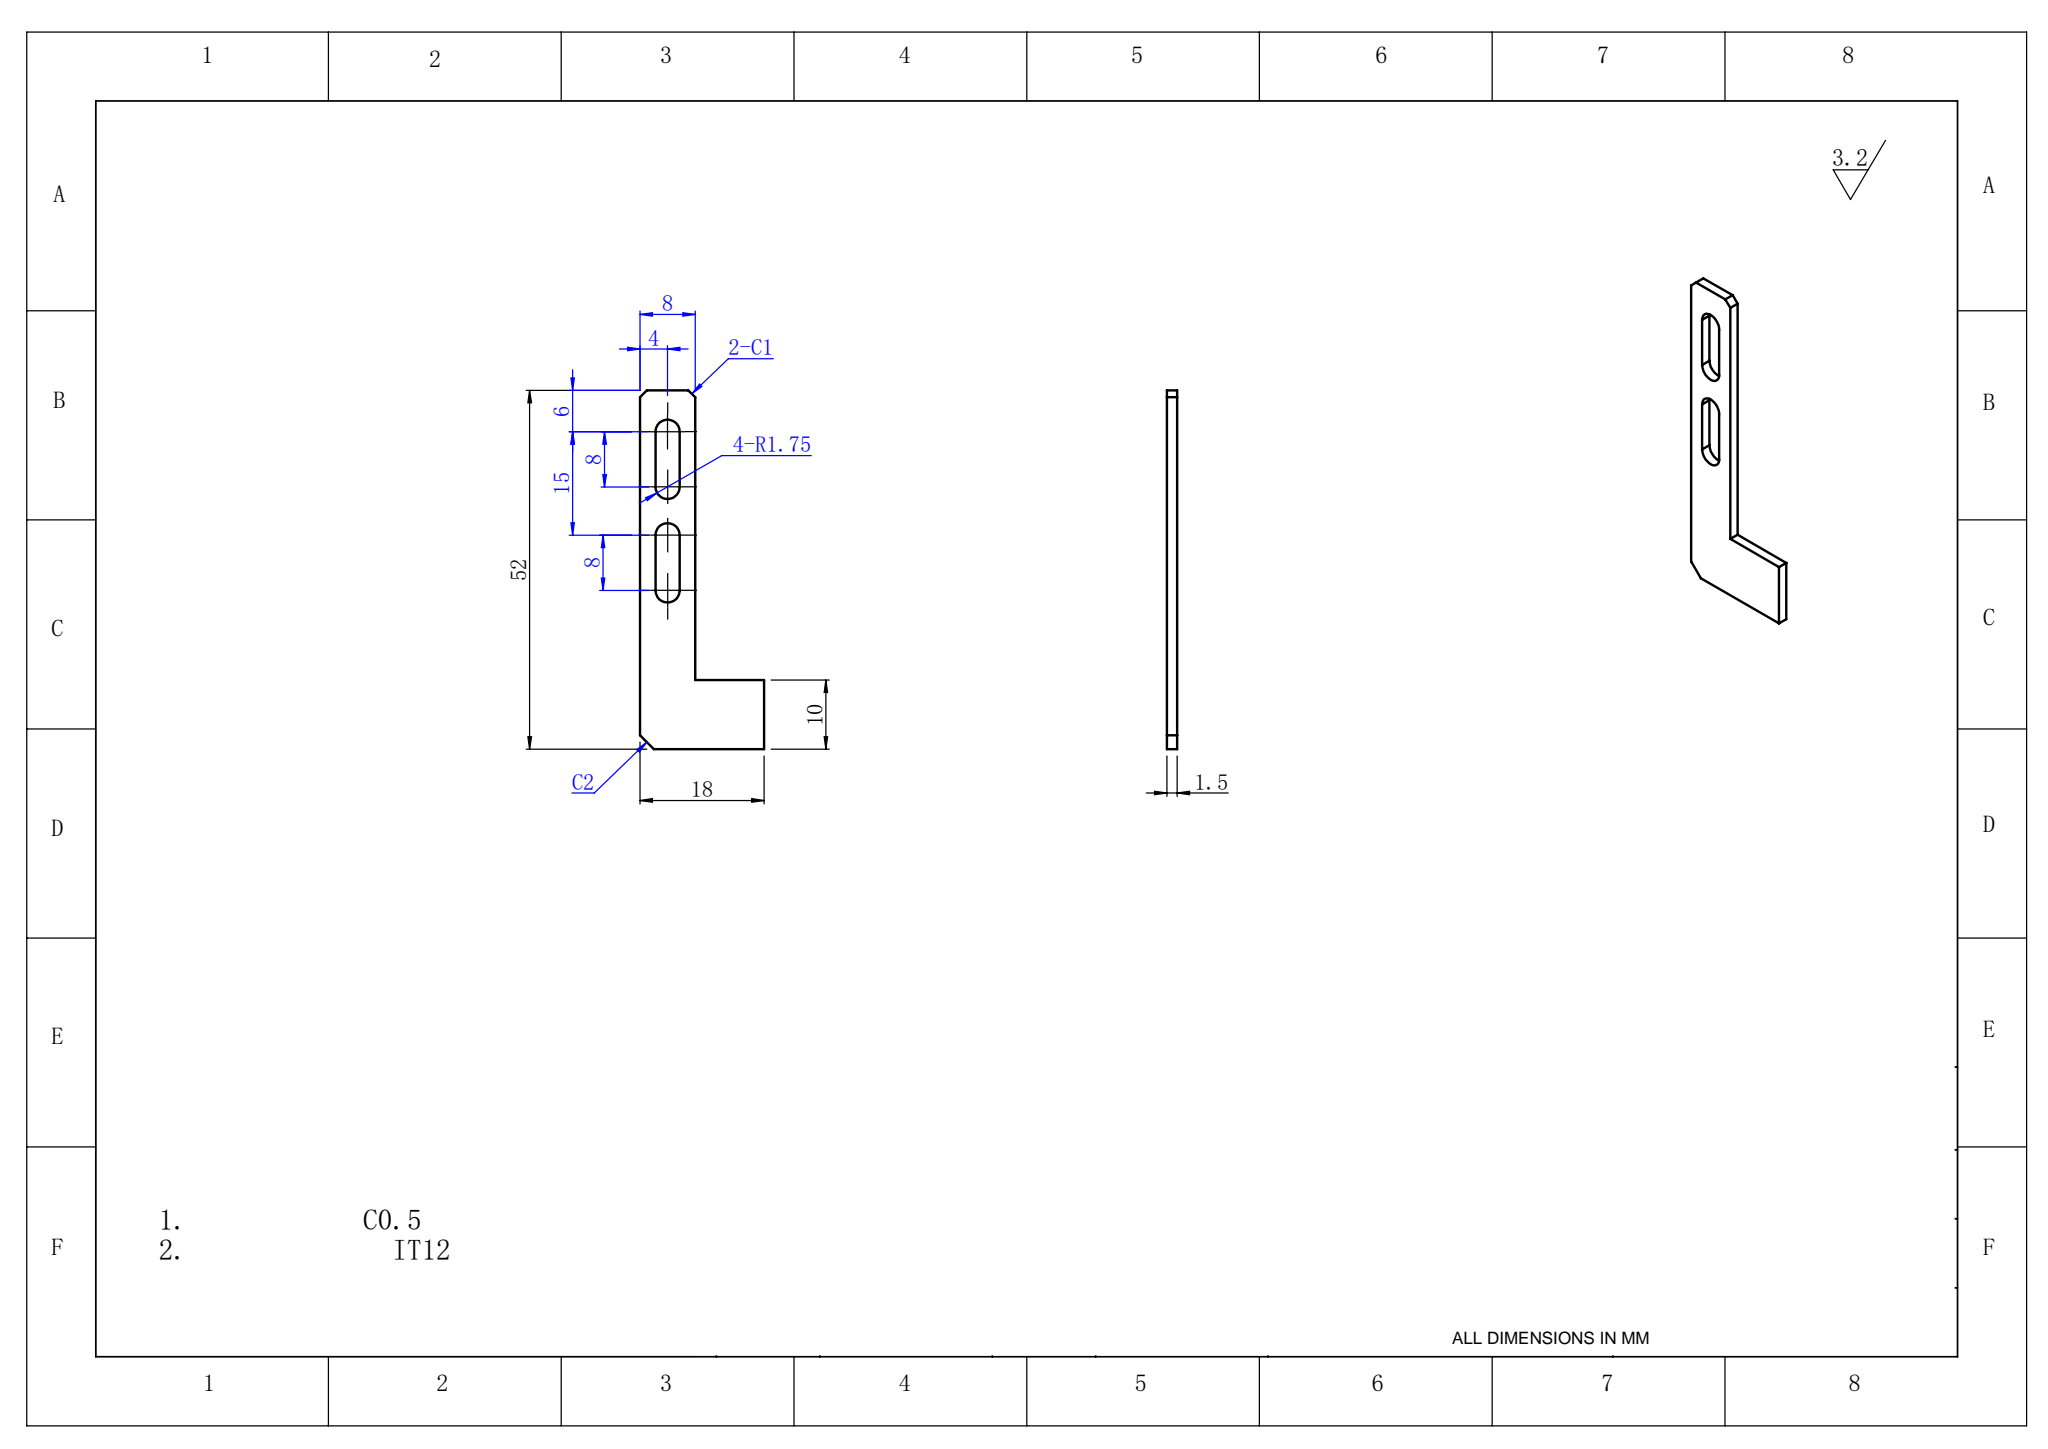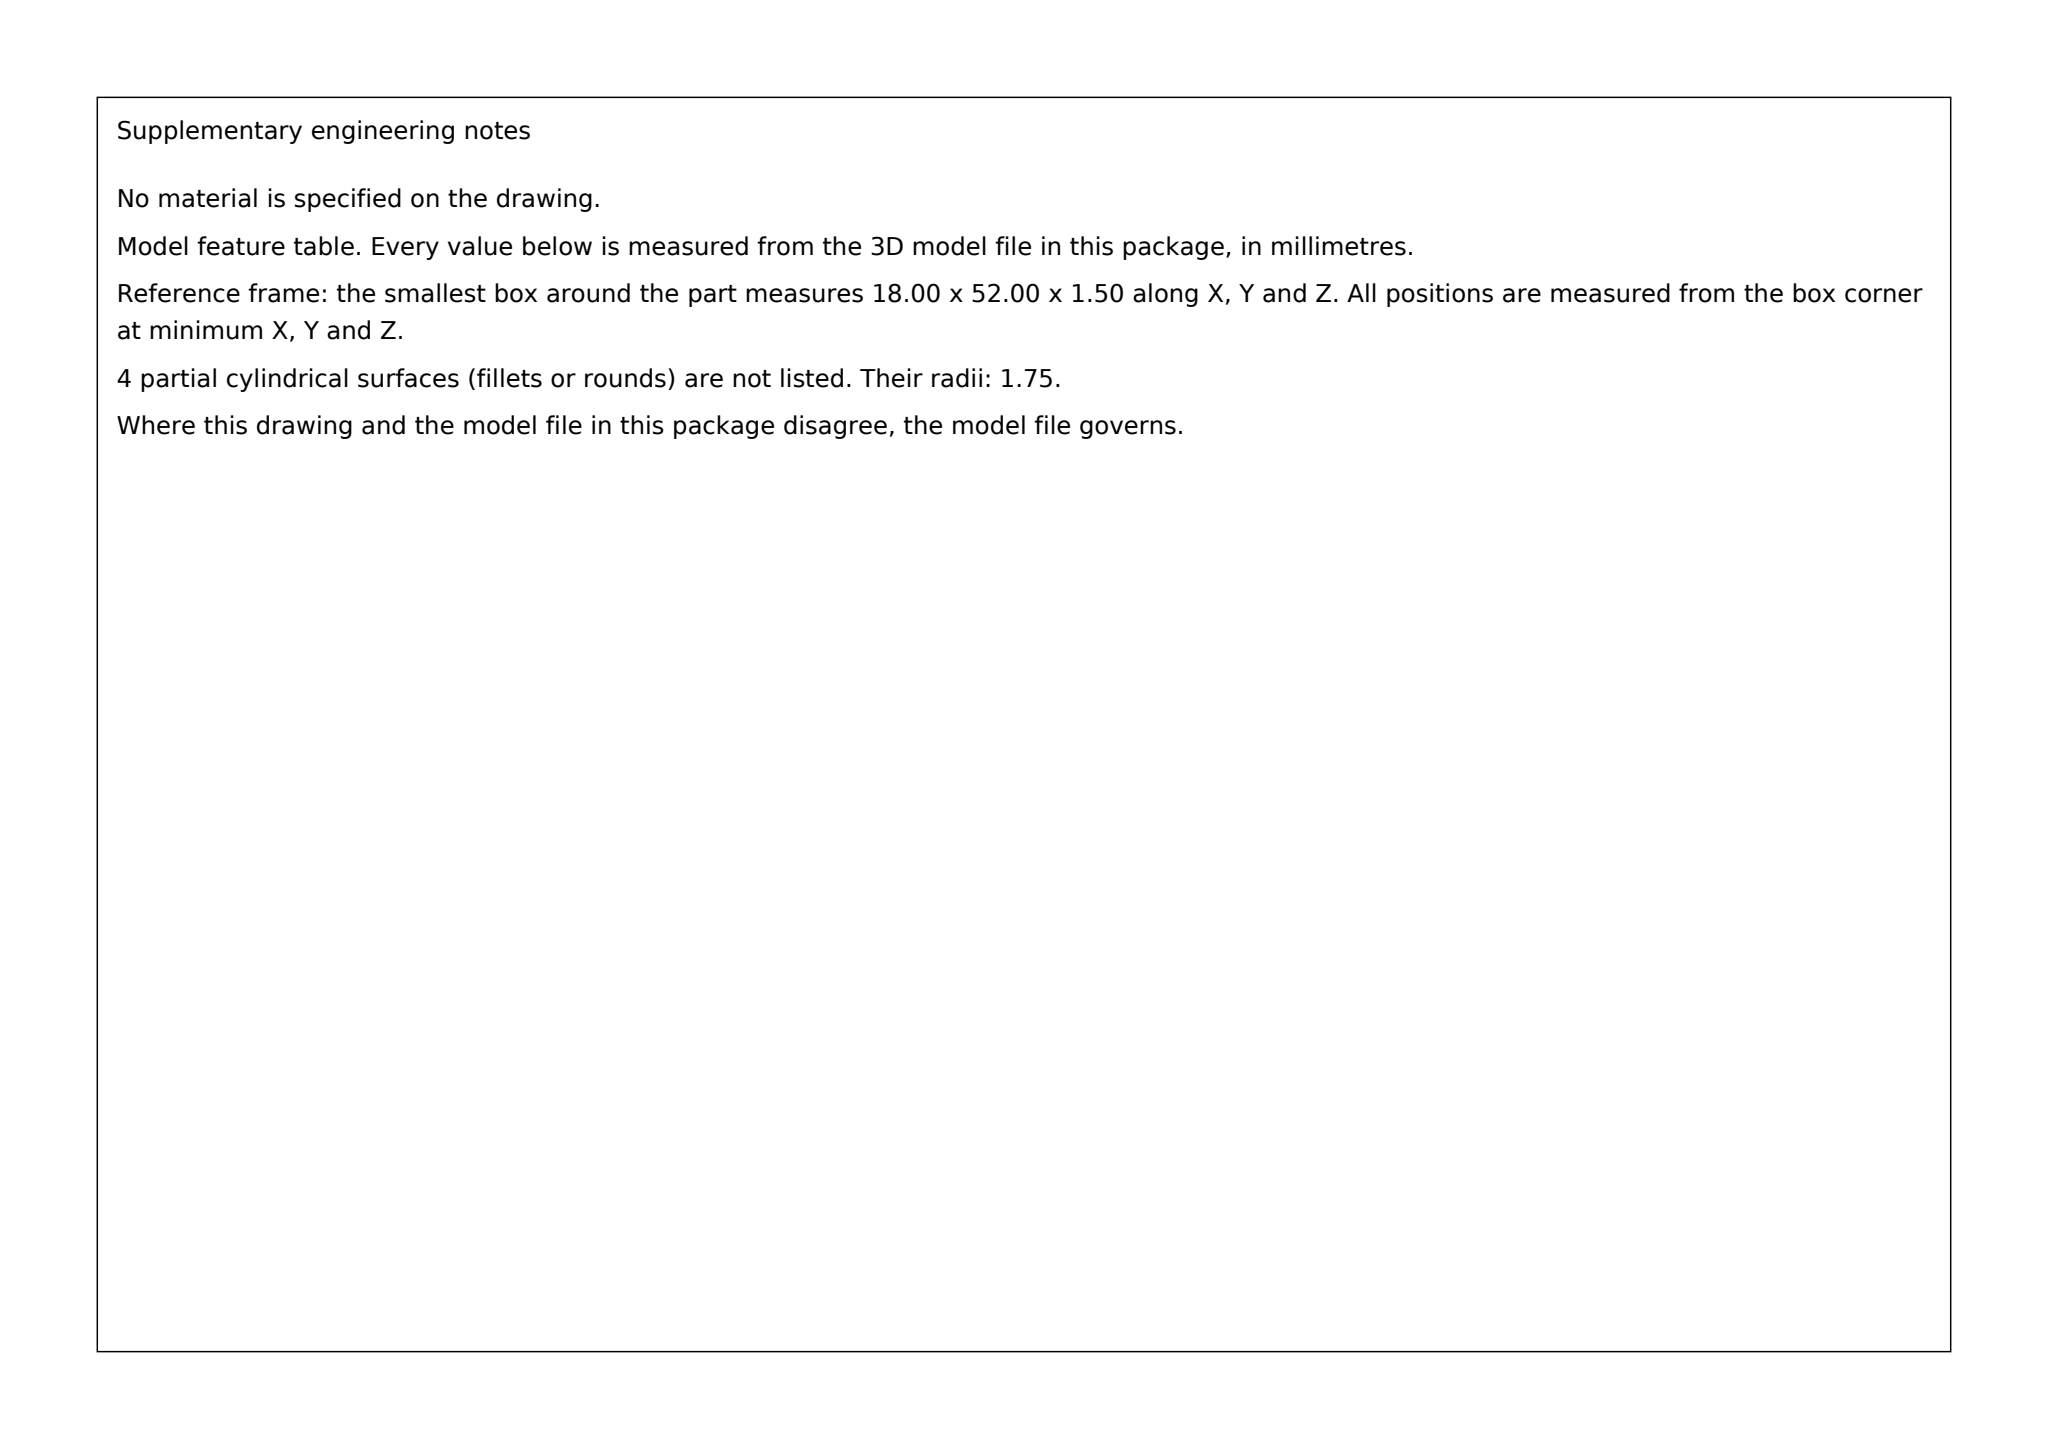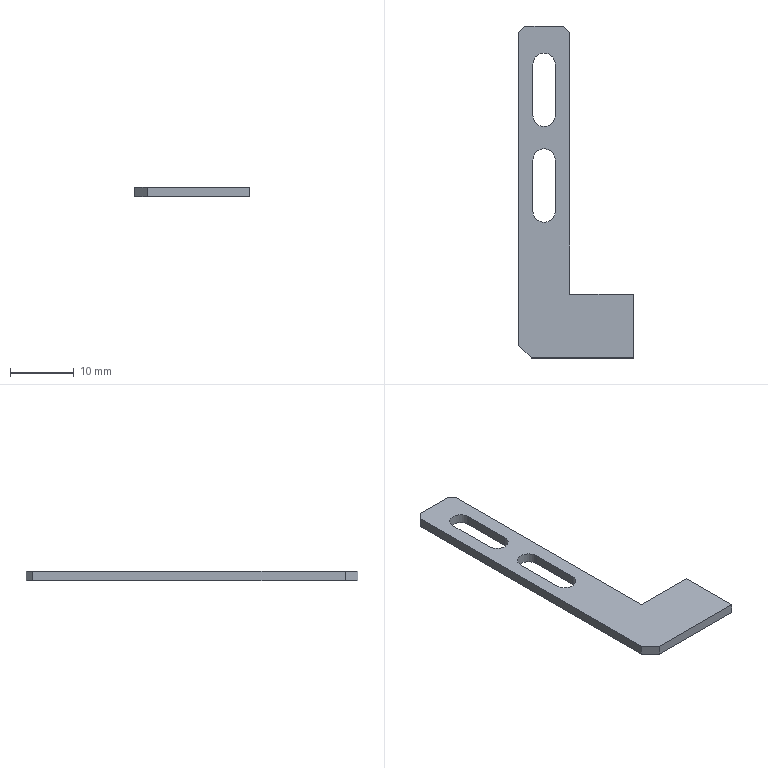Part | SolidWorks | mm | 1 solid | 19 faces | box 18 x 52 x 1.5 mm | volume 657 mm3 | plane 15 | cylinder 4 | commonest cylinder face diameters 3.5 x4
STEP:
#1=CARTESIAN_POINT('',(8.,-42.,1.5));
#2=VERTEX_POINT('',#1);
#3=CARTESIAN_POINT('',(8.,-42.,0.));
#4=VERTEX_POINT('',#3);
#5=CARTESIAN_POINT('',(8.,-42.,0.));
#6=DIRECTION('',(0.,0.,-1.));
#7=VECTOR('',#6,1000.);
#8=LINE('',#5,#7);
#9=EDGE_CURVE('',#2,#4,#8,.T.);
#10=ORIENTED_EDGE('',*,*,#9,.F.);
#11=CARTESIAN_POINT('',(18.,-42.,1.5));
#12=VERTEX_POINT('',#11);
#13=CARTESIAN_POINT('',(0.,-42.,1.5));
#14=DIRECTION('',(-1.,0.,0.));
#15=VECTOR('',#14,1000.);
#16=LINE('',#13,#15);
#17=EDGE_CURVE('',#12,#2,#16,.T.);
#18=ORIENTED_EDGE('',*,*,#17,.F.);
#19=CARTESIAN_POINT('',(18.,-42.,0.));
#20=VERTEX_POINT('',#19);
#21=CARTESIAN_POINT('',(18.,-42.,0.));
#22=DIRECTION('',(0.,0.,-1.));
#23=VECTOR('',#22,1000.);
#24=LINE('',#21,#23);
#25=EDGE_CURVE('',#12,#20,#24,.T.);
#26=ORIENTED_EDGE('',*,*,#25,.T.);
#27=CARTESIAN_POINT('',(18.,-42.,0.));
#28=DIRECTION('',(-1.,0.,0.));
#29=VECTOR('',#28,1000.);
#30=LINE('',#27,#29);
#31=EDGE_CURVE('',#20,#4,#30,.T.);
#32=ORIENTED_EDGE('',*,*,#31,.T.);
#33=EDGE_LOOP('',(#10,#18,#26,#32));
#34=FACE_OUTER_BOUND('',#33,.T.);
#35=CARTESIAN_POINT('',(18.,-42.,0.));
#36=DIRECTION('',(0.,1.,0.));
#37=DIRECTION('',(-1.,0.,0.));
#38=AXIS2_PLACEMENT_3D('',#35,#36,#37);
#39=PLANE('',#38);
#40=ADVANCED_FACE('',(#34),#39,.T.);
#41=ORIENTED_EDGE('',*,*,#25,.F.);
#42=CARTESIAN_POINT('',(18.,-52.,1.5));
#43=VERTEX_POINT('',#42);
#44=CARTESIAN_POINT('',(18.,0.,1.5));
#45=DIRECTION('',(0.,1.,0.));
#46=VECTOR('',#45,1000.);
#47=LINE('',#44,#46);
#48=EDGE_CURVE('',#43,#12,#47,.T.);
#49=ORIENTED_EDGE('',*,*,#48,.F.);
#50=CARTESIAN_POINT('',(18.,-52.,0.));
#51=VERTEX_POINT('',#50);
#52=CARTESIAN_POINT('',(18.,-52.,0.));
#53=DIRECTION('',(0.,0.,-1.));
#54=VECTOR('',#53,1000.);
#55=LINE('',#52,#54);
#56=EDGE_CURVE('',#43,#51,#55,.T.);
#57=ORIENTED_EDGE('',*,*,#56,.T.);
#58=CARTESIAN_POINT('',(18.,-52.,0.));
#59=DIRECTION('',(0.,1.,0.));
#60=VECTOR('',#59,1000.);
#61=LINE('',#58,#60);
#62=EDGE_CURVE('',#51,#20,#61,.T.);
#63=ORIENTED_EDGE('',*,*,#62,.T.);
#64=EDGE_LOOP('',(#41,#49,#57,#63));
#65=FACE_OUTER_BOUND('',#64,.T.);
#66=CARTESIAN_POINT('',(18.,-52.,0.));
#67=DIRECTION('',(1.,0.,0.));
#68=DIRECTION('',(0.,1.,0.));
#69=AXIS2_PLACEMENT_3D('',#66,#67,#68);
#70=PLANE('',#69);
#71=ADVANCED_FACE('',(#65),#70,.T.);
#72=CARTESIAN_POINT('',(2.,-52.,1.5));
#73=VERTEX_POINT('',#72);
#74=CARTESIAN_POINT('',(0.,-52.,1.5));
#75=DIRECTION('',(1.,0.,0.));
#76=VECTOR('',#75,1000.);
#77=LINE('',#74,#76);
#78=EDGE_CURVE('',#73,#43,#77,.T.);
#79=ORIENTED_EDGE('',*,*,#78,.F.);
#80=CARTESIAN_POINT('',(2.,-52.,0.));
#81=VERTEX_POINT('',#80);
#82=CARTESIAN_POINT('',(2.,-52.,0.));
#83=DIRECTION('',(0.,0.,-1.));
#84=VECTOR('',#83,1000.);
#85=LINE('',#82,#84);
#86=EDGE_CURVE('',#73,#81,#85,.T.);
#87=ORIENTED_EDGE('',*,*,#86,.T.);
#88=CARTESIAN_POINT('',(0.,-52.,0.));
#89=DIRECTION('',(1.,0.,0.));
#90=VECTOR('',#89,1000.);
#91=LINE('',#88,#90);
#92=EDGE_CURVE('',#81,#51,#91,.T.);
#93=ORIENTED_EDGE('',*,*,#92,.T.);
#94=ORIENTED_EDGE('',*,*,#56,.F.);
#95=EDGE_LOOP('',(#79,#87,#93,#94));
#96=FACE_OUTER_BOUND('',#95,.T.);
#97=CARTESIAN_POINT('',(0.,-52.,0.));
#98=DIRECTION('',(0.,-1.,0.));
#99=DIRECTION('',(1.,0.,0.));
#100=AXIS2_PLACEMENT_3D('',#97,#98,#99);
#101=PLANE('',#100);
#102=ADVANCED_FACE('',(#96),#101,.T.);
#103=CARTESIAN_POINT('',(0.,-1.,0.));
#104=VERTEX_POINT('',#103);
#105=CARTESIAN_POINT('',(0.,-50.,0.));
#106=VERTEX_POINT('',#105);
#107=CARTESIAN_POINT('',(0.,0.,0.));
#108=DIRECTION('',(0.,-1.,0.));
#109=VECTOR('',#108,1000.);
#110=LINE('',#107,#109);
#111=EDGE_CURVE('',#104,#106,#110,.T.);
#112=ORIENTED_EDGE('',*,*,#111,.T.);
#113=CARTESIAN_POINT('',(0.,-50.,1.5));
#114=VERTEX_POINT('',#113);
#115=CARTESIAN_POINT('',(0.,-50.,0.));
#116=DIRECTION('',(0.,0.,1.));
#117=VECTOR('',#116,1000.);
#118=LINE('',#115,#117);
#119=EDGE_CURVE('',#106,#114,#118,.T.);
#120=ORIENTED_EDGE('',*,*,#119,.T.);
#121=CARTESIAN_POINT('',(0.,-1.,1.5));
#122=VERTEX_POINT('',#121);
#123=CARTESIAN_POINT('',(0.,0.,1.5));
#124=DIRECTION('',(0.,-1.,0.));
#125=VECTOR('',#124,1000.);
#126=LINE('',#123,#125);
#127=EDGE_CURVE('',#122,#114,#126,.T.);
#128=ORIENTED_EDGE('',*,*,#127,.F.);
#129=CARTESIAN_POINT('',(0.,-1.,0.));
#130=DIRECTION('',(0.,0.,-1.));
#131=VECTOR('',#130,1000.);
#132=LINE('',#129,#131);
#133=EDGE_CURVE('',#122,#104,#132,.T.);
#134=ORIENTED_EDGE('',*,*,#133,.T.);
#135=EDGE_LOOP('',(#112,#120,#128,#134));
#136=FACE_OUTER_BOUND('',#135,.T.);
#137=CARTESIAN_POINT('',(0.,0.,0.));
#138=DIRECTION('',(-1.,-0.,0.));
#139=DIRECTION('',(0.,-1.,0.));
#140=AXIS2_PLACEMENT_3D('',#137,#138,#139);
#141=PLANE('',#140);
#142=ADVANCED_FACE('',(#136),#141,.T.);
#143=CARTESIAN_POINT('',(7.,-0.,1.5));
#144=VERTEX_POINT('',#143);
#145=CARTESIAN_POINT('',(1.,-0.,1.5));
#146=VERTEX_POINT('',#145);
#147=CARTESIAN_POINT('',(0.,-0.,1.5));
#148=DIRECTION('',(-1.,0.,0.));
#149=VECTOR('',#148,1000.);
#150=LINE('',#147,#149);
#151=EDGE_CURVE('',#144,#146,#150,.T.);
#152=ORIENTED_EDGE('',*,*,#151,.F.);
#153=CARTESIAN_POINT('',(7.,-0.,0.));
#154=VERTEX_POINT('',#153);
#155=CARTESIAN_POINT('',(7.,-0.,0.));
#156=DIRECTION('',(0.,0.,-1.));
#157=VECTOR('',#156,1000.);
#158=LINE('',#155,#157);
#159=EDGE_CURVE('',#144,#154,#158,.T.);
#160=ORIENTED_EDGE('',*,*,#159,.T.);
#161=CARTESIAN_POINT('',(1.,-0.,0.));
#162=VERTEX_POINT('',#161);
#163=CARTESIAN_POINT('',(8.,-0.,0.));
#164=DIRECTION('',(-1.,0.,0.));
#165=VECTOR('',#164,1000.);
#166=LINE('',#163,#165);
#167=EDGE_CURVE('',#154,#162,#166,.T.);
#168=ORIENTED_EDGE('',*,*,#167,.T.);
#169=CARTESIAN_POINT('',(1.,-0.,0.));
#170=DIRECTION('',(0.,0.,1.));
#171=VECTOR('',#170,1000.);
#172=LINE('',#169,#171);
#173=EDGE_CURVE('',#162,#146,#172,.T.);
#174=ORIENTED_EDGE('',*,*,#173,.T.);
#175=EDGE_LOOP('',(#152,#160,#168,#174));
#176=FACE_OUTER_BOUND('',#175,.T.);
#177=CARTESIAN_POINT('',(8.,-0.,0.));
#178=DIRECTION('',(0.,1.,0.));
#179=DIRECTION('',(-1.,0.,0.));
#180=AXIS2_PLACEMENT_3D('',#177,#178,#179);
#181=PLANE('',#180);
#182=ADVANCED_FACE('',(#176),#181,.T.);
#183=CARTESIAN_POINT('',(2.25,-6.,1.5));
#184=VERTEX_POINT('',#183);
#185=CARTESIAN_POINT('',(2.25,-6.,0.));
#186=VERTEX_POINT('',#185);
#187=CARTESIAN_POINT('',(2.25,-6.,0.));
#188=DIRECTION('',(0.,0.,-1.));
#189=VECTOR('',#188,1000.);
#190=LINE('',#187,#189);
#191=EDGE_CURVE('',#184,#186,#190,.T.);
#192=ORIENTED_EDGE('',*,*,#191,.F.);
#193=CARTESIAN_POINT('',(2.25,-14.,1.5));
#194=VERTEX_POINT('',#193);
#195=CARTESIAN_POINT('',(2.25,0.,1.5));
#196=DIRECTION('',(0.,-1.,0.));
#197=VECTOR('',#196,1000.);
#198=LINE('',#195,#197);
#199=EDGE_CURVE('',#184,#194,#198,.T.);
#200=ORIENTED_EDGE('',*,*,#199,.T.);
#201=CARTESIAN_POINT('',(2.25,-14.,0.));
#202=VERTEX_POINT('',#201);
#203=CARTESIAN_POINT('',(2.25,-14.,0.));
#204=DIRECTION('',(0.,0.,-1.));
#205=VECTOR('',#204,1000.);
#206=LINE('',#203,#205);
#207=EDGE_CURVE('',#194,#202,#206,.T.);
#208=ORIENTED_EDGE('',*,*,#207,.T.);
#209=CARTESIAN_POINT('',(2.25,-6.,0.));
#210=DIRECTION('',(0.,-1.,0.));
#211=VECTOR('',#210,1000.);
#212=LINE('',#209,#211);
#213=EDGE_CURVE('',#186,#202,#212,.T.);
#214=ORIENTED_EDGE('',*,*,#213,.F.);
#215=EDGE_LOOP('',(#192,#200,#208,#214));
#216=FACE_OUTER_BOUND('',#215,.T.);
#217=CARTESIAN_POINT('',(2.25,-6.,0.));
#218=DIRECTION('',(-1.,-0.,0.));
#219=DIRECTION('',(0.,-1.,0.));
#220=AXIS2_PLACEMENT_3D('',#217,#218,#219);
#221=PLANE('',#220);
#222=ADVANCED_FACE('',(#216),#221,.F.);
#223=ORIENTED_EDGE('',*,*,#207,.F.);
#224=CARTESIAN_POINT('',(5.75,-14.,1.5));
#225=VERTEX_POINT('',#224);
#226=CARTESIAN_POINT('',(4.,-14.,1.5));
#227=DIRECTION('',(0.,0.,1.));
#228=DIRECTION('',(1.,0.,0.));
#229=AXIS2_PLACEMENT_3D('',#226,#227,#228);
#230=CIRCLE('',#229,1.75);
#231=EDGE_CURVE('',#194,#225,#230,.T.);
#232=ORIENTED_EDGE('',*,*,#231,.T.);
#233=CARTESIAN_POINT('',(5.75,-14.,0.));
#234=VERTEX_POINT('',#233);
#235=CARTESIAN_POINT('',(5.75,-14.,0.));
#236=DIRECTION('',(0.,0.,-1.));
#237=VECTOR('',#236,1000.);
#238=LINE('',#235,#237);
#239=EDGE_CURVE('',#225,#234,#238,.T.);
#240=ORIENTED_EDGE('',*,*,#239,.T.);
#241=CARTESIAN_POINT('',(4.,-14.,0.));
#242=DIRECTION('',(0.,0.,1.));
#243=DIRECTION('',(1.,0.,0.));
#244=AXIS2_PLACEMENT_3D('',#241,#242,#243);
#245=CIRCLE('',#244,1.75);
#246=EDGE_CURVE('',#202,#234,#245,.T.);
#247=ORIENTED_EDGE('',*,*,#246,.F.);
#248=EDGE_LOOP('',(#223,#232,#240,#247));
#249=FACE_OUTER_BOUND('',#248,.T.);
#250=CARTESIAN_POINT('',(4.,-14.,0.));
#251=DIRECTION('',(0.,0.,1.));
#252=DIRECTION('',(1.,0.,0.));
#253=AXIS2_PLACEMENT_3D('',#250,#251,#252);
#254=CYLINDRICAL_SURFACE('',#253,1.75);
#255=ADVANCED_FACE('',(#249),#254,.F.);
#256=ORIENTED_EDGE('',*,*,#239,.F.);
#257=CARTESIAN_POINT('',(5.75,-6.,1.5));
#258=VERTEX_POINT('',#257);
#259=CARTESIAN_POINT('',(5.75,0.,1.5));
#260=DIRECTION('',(0.,1.,0.));
#261=VECTOR('',#260,1000.);
#262=LINE('',#259,#261);
#263=EDGE_CURVE('',#225,#258,#262,.T.);
#264=ORIENTED_EDGE('',*,*,#263,.T.);
#265=CARTESIAN_POINT('',(5.75,-6.,0.));
#266=VERTEX_POINT('',#265);
#267=CARTESIAN_POINT('',(5.75,-6.,0.));
#268=DIRECTION('',(0.,0.,-1.));
#269=VECTOR('',#268,1000.);
#270=LINE('',#267,#269);
#271=EDGE_CURVE('',#258,#266,#270,.T.);
#272=ORIENTED_EDGE('',*,*,#271,.T.);
#273=CARTESIAN_POINT('',(5.75,-6.,0.));
#274=DIRECTION('',(-0.,1.,0.));
#275=VECTOR('',#274,1000.);
#276=LINE('',#273,#275);
#277=EDGE_CURVE('',#234,#266,#276,.T.);
#278=ORIENTED_EDGE('',*,*,#277,.F.);
#279=EDGE_LOOP('',(#256,#264,#272,#278));
#280=FACE_OUTER_BOUND('',#279,.T.);
#281=CARTESIAN_POINT('',(5.75,-6.,0.));
#282=DIRECTION('',(1.,0.,0.));
#283=DIRECTION('',(-0.,1.,0.));
#284=AXIS2_PLACEMENT_3D('',#281,#282,#283);
#285=PLANE('',#284);
#286=ADVANCED_FACE('',(#280),#285,.F.);
#287=CARTESIAN_POINT('',(2.25,-21.,1.5));
#288=VERTEX_POINT('',#287);
#289=CARTESIAN_POINT('',(2.25,-21.,0.));
#290=VERTEX_POINT('',#289);
#291=CARTESIAN_POINT('',(2.25,-21.,0.));
#292=DIRECTION('',(0.,0.,-1.));
#293=VECTOR('',#292,1000.);
#294=LINE('',#291,#293);
#295=EDGE_CURVE('',#288,#290,#294,.T.);
#296=ORIENTED_EDGE('',*,*,#295,.F.);
#297=CARTESIAN_POINT('',(2.25,-29.,1.5));
#298=VERTEX_POINT('',#297);
#299=CARTESIAN_POINT('',(2.25,0.,1.5));
#300=DIRECTION('',(0.,-1.,0.));
#301=VECTOR('',#300,1000.);
#302=LINE('',#299,#301);
#303=EDGE_CURVE('',#288,#298,#302,.T.);
#304=ORIENTED_EDGE('',*,*,#303,.T.);
#305=CARTESIAN_POINT('',(2.25,-29.,0.));
#306=VERTEX_POINT('',#305);
#307=CARTESIAN_POINT('',(2.25,-29.,0.));
#308=DIRECTION('',(0.,0.,-1.));
#309=VECTOR('',#308,1000.);
#310=LINE('',#307,#309);
#311=EDGE_CURVE('',#298,#306,#310,.T.);
#312=ORIENTED_EDGE('',*,*,#311,.T.);
#313=CARTESIAN_POINT('',(2.25,-21.,0.));
#314=DIRECTION('',(0.,-1.,0.));
#315=VECTOR('',#314,1000.);
#316=LINE('',#313,#315);
#317=EDGE_CURVE('',#290,#306,#316,.T.);
#318=ORIENTED_EDGE('',*,*,#317,.F.);
#319=EDGE_LOOP('',(#296,#304,#312,#318));
#320=FACE_OUTER_BOUND('',#319,.T.);
#321=CARTESIAN_POINT('',(2.25,-21.,0.));
#322=DIRECTION('',(-1.,-0.,0.));
#323=DIRECTION('',(0.,-1.,0.));
#324=AXIS2_PLACEMENT_3D('',#321,#322,#323);
#325=PLANE('',#324);
#326=ADVANCED_FACE('',(#320),#325,.F.);
#327=ORIENTED_EDGE('',*,*,#311,.F.);
#328=CARTESIAN_POINT('',(5.75,-29.,1.5));
#329=VERTEX_POINT('',#328);
#330=CARTESIAN_POINT('',(4.,-29.,1.5));
#331=DIRECTION('',(0.,0.,1.));
#332=DIRECTION('',(1.,0.,0.));
#333=AXIS2_PLACEMENT_3D('',#330,#331,#332);
#334=CIRCLE('',#333,1.75);
#335=EDGE_CURVE('',#298,#329,#334,.T.);
#336=ORIENTED_EDGE('',*,*,#335,.T.);
#337=CARTESIAN_POINT('',(5.75,-29.,0.));
#338=VERTEX_POINT('',#337);
#339=CARTESIAN_POINT('',(5.75,-29.,0.));
#340=DIRECTION('',(0.,0.,-1.));
#341=VECTOR('',#340,1000.);
#342=LINE('',#339,#341);
#343=EDGE_CURVE('',#329,#338,#342,.T.);
#344=ORIENTED_EDGE('',*,*,#343,.T.);
#345=CARTESIAN_POINT('',(4.,-29.,0.));
#346=DIRECTION('',(0.,0.,1.));
#347=DIRECTION('',(1.,0.,0.));
#348=AXIS2_PLACEMENT_3D('',#345,#346,#347);
#349=CIRCLE('',#348,1.75);
#350=EDGE_CURVE('',#306,#338,#349,.T.);
#351=ORIENTED_EDGE('',*,*,#350,.F.);
#352=EDGE_LOOP('',(#327,#336,#344,#351));
#353=FACE_OUTER_BOUND('',#352,.T.);
#354=CARTESIAN_POINT('',(4.,-29.,0.));
#355=DIRECTION('',(0.,0.,1.));
#356=DIRECTION('',(1.,0.,0.));
#357=AXIS2_PLACEMENT_3D('',#354,#355,#356);
#358=CYLINDRICAL_SURFACE('',#357,1.75);
#359=ADVANCED_FACE('',(#353),#358,.F.);
#360=ORIENTED_EDGE('',*,*,#343,.F.);
#361=CARTESIAN_POINT('',(5.75,-21.,1.5));
#362=VERTEX_POINT('',#361);
#363=CARTESIAN_POINT('',(5.75,0.,1.5));
#364=DIRECTION('',(0.,1.,0.));
#365=VECTOR('',#364,1000.);
#366=LINE('',#363,#365);
#367=EDGE_CURVE('',#329,#362,#366,.T.);
#368=ORIENTED_EDGE('',*,*,#367,.T.);
#369=CARTESIAN_POINT('',(5.75,-21.,0.));
#370=VERTEX_POINT('',#369);
#371=CARTESIAN_POINT('',(5.75,-21.,0.));
#372=DIRECTION('',(0.,0.,-1.));
#373=VECTOR('',#372,1000.);
#374=LINE('',#371,#373);
#375=EDGE_CURVE('',#362,#370,#374,.T.);
#376=ORIENTED_EDGE('',*,*,#375,.T.);
#377=CARTESIAN_POINT('',(5.75,-21.,0.));
#378=DIRECTION('',(-0.,1.,0.));
#379=VECTOR('',#378,1000.);
#380=LINE('',#377,#379);
#381=EDGE_CURVE('',#338,#370,#380,.T.);
#382=ORIENTED_EDGE('',*,*,#381,.F.);
#383=EDGE_LOOP('',(#360,#368,#376,#382));
#384=FACE_OUTER_BOUND('',#383,.T.);
#385=CARTESIAN_POINT('',(5.75,-21.,0.));
#386=DIRECTION('',(1.,0.,0.));
#387=DIRECTION('',(-0.,1.,0.));
#388=AXIS2_PLACEMENT_3D('',#385,#386,#387);
#389=PLANE('',#388);
#390=ADVANCED_FACE('',(#384),#389,.F.);
#391=CARTESIAN_POINT('',(4.,-21.,1.5));
#392=DIRECTION('',(0.,0.,1.));
#393=DIRECTION('',(1.,0.,0.));
#394=AXIS2_PLACEMENT_3D('',#391,#392,#393);
#395=CIRCLE('',#394,1.75);
#396=EDGE_CURVE('',#362,#288,#395,.T.);
#397=ORIENTED_EDGE('',*,*,#396,.T.);
#398=ORIENTED_EDGE('',*,*,#295,.T.);
#399=CARTESIAN_POINT('',(4.,-21.,0.));
#400=DIRECTION('',(0.,0.,1.));
#401=DIRECTION('',(1.,0.,0.));
#402=AXIS2_PLACEMENT_3D('',#399,#400,#401);
#403=CIRCLE('',#402,1.75);
#404=EDGE_CURVE('',#370,#290,#403,.T.);
#405=ORIENTED_EDGE('',*,*,#404,.F.);
#406=ORIENTED_EDGE('',*,*,#375,.F.);
#407=EDGE_LOOP('',(#397,#398,#405,#406));
#408=FACE_OUTER_BOUND('',#407,.T.);
#409=CARTESIAN_POINT('',(4.,-21.,0.));
#410=DIRECTION('',(0.,0.,1.));
#411=DIRECTION('',(1.,0.,0.));
#412=AXIS2_PLACEMENT_3D('',#409,#410,#411);
#413=CYLINDRICAL_SURFACE('',#412,1.75);
#414=ADVANCED_FACE('',(#408),#413,.F.);
#415=CARTESIAN_POINT('',(4.,-6.,1.5));
#416=DIRECTION('',(0.,0.,1.));
#417=DIRECTION('',(1.,0.,0.));
#418=AXIS2_PLACEMENT_3D('',#415,#416,#417);
#419=CIRCLE('',#418,1.75);
#420=EDGE_CURVE('',#258,#184,#419,.T.);
#421=ORIENTED_EDGE('',*,*,#420,.T.);
#422=ORIENTED_EDGE('',*,*,#191,.T.);
#423=CARTESIAN_POINT('',(4.,-6.,0.));
#424=DIRECTION('',(0.,0.,1.));
#425=DIRECTION('',(1.,0.,0.));
#426=AXIS2_PLACEMENT_3D('',#423,#424,#425);
#427=CIRCLE('',#426,1.75);
#428=EDGE_CURVE('',#266,#186,#427,.T.);
#429=ORIENTED_EDGE('',*,*,#428,.F.);
#430=ORIENTED_EDGE('',*,*,#271,.F.);
#431=EDGE_LOOP('',(#421,#422,#429,#430));
#432=FACE_OUTER_BOUND('',#431,.T.);
#433=CARTESIAN_POINT('',(4.,-6.,0.));
#434=DIRECTION('',(0.,0.,1.));
#435=DIRECTION('',(1.,0.,0.));
#436=AXIS2_PLACEMENT_3D('',#433,#434,#435);
#437=CYLINDRICAL_SURFACE('',#436,1.75);
#438=ADVANCED_FACE('',(#432),#437,.F.);
#439=CARTESIAN_POINT('',(8.,-1.,0.));
#440=VERTEX_POINT('',#439);
#441=CARTESIAN_POINT('',(8.,-42.,0.));
#442=DIRECTION('',(0.,1.,0.));
#443=VECTOR('',#442,1000.);
#444=LINE('',#441,#443);
#445=EDGE_CURVE('',#4,#440,#444,.T.);
#446=ORIENTED_EDGE('',*,*,#445,.T.);
#447=CARTESIAN_POINT('',(8.,-1.,1.5));
#448=VERTEX_POINT('',#447);
#449=CARTESIAN_POINT('',(8.,-1.,0.));
#450=DIRECTION('',(0.,0.,1.));
#451=VECTOR('',#450,1000.);
#452=LINE('',#449,#451);
#453=EDGE_CURVE('',#440,#448,#452,.T.);
#454=ORIENTED_EDGE('',*,*,#453,.T.);
#455=CARTESIAN_POINT('',(8.,0.,1.5));
#456=DIRECTION('',(0.,1.,0.));
#457=VECTOR('',#456,1000.);
#458=LINE('',#455,#457);
#459=EDGE_CURVE('',#2,#448,#458,.T.);
#460=ORIENTED_EDGE('',*,*,#459,.F.);
#461=ORIENTED_EDGE('',*,*,#9,.T.);
#462=EDGE_LOOP('',(#446,#454,#460,#461));
#463=FACE_OUTER_BOUND('',#462,.T.);
#464=CARTESIAN_POINT('',(8.,-42.,0.));
#465=DIRECTION('',(1.,0.,0.));
#466=DIRECTION('',(0.,1.,0.));
#467=AXIS2_PLACEMENT_3D('',#464,#465,#466);
#468=PLANE('',#467);
#469=ADVANCED_FACE('',(#463),#468,.T.);
#470=ORIENTED_EDGE('',*,*,#381,.T.);
#471=ORIENTED_EDGE('',*,*,#404,.T.);
#472=ORIENTED_EDGE('',*,*,#317,.T.);
#473=ORIENTED_EDGE('',*,*,#350,.T.);
#474=EDGE_LOOP('',(#470,#471,#472,#473));
#475=FACE_BOUND('',#474,.T.);
#476=ORIENTED_EDGE('',*,*,#277,.T.);
#477=ORIENTED_EDGE('',*,*,#428,.T.);
#478=ORIENTED_EDGE('',*,*,#213,.T.);
#479=ORIENTED_EDGE('',*,*,#246,.T.);
#480=EDGE_LOOP('',(#476,#477,#478,#479));
#481=FACE_BOUND('',#480,.T.);
#482=ORIENTED_EDGE('',*,*,#92,.F.);
#483=CARTESIAN_POINT('',(2.,-52.,0.));
#484=DIRECTION('',(-0.7071,0.7071,0.));
#485=VECTOR('',#484,1000.);
#486=LINE('',#483,#485);
#487=EDGE_CURVE('',#81,#106,#486,.T.);
#488=ORIENTED_EDGE('',*,*,#487,.T.);
#489=ORIENTED_EDGE('',*,*,#111,.F.);
#490=CARTESIAN_POINT('',(0.,-1.,0.));
#491=DIRECTION('',(0.7071,0.7071,0.));
#492=VECTOR('',#491,1000.);
#493=LINE('',#490,#492);
#494=EDGE_CURVE('',#104,#162,#493,.T.);
#495=ORIENTED_EDGE('',*,*,#494,.T.);
#496=ORIENTED_EDGE('',*,*,#167,.F.);
#497=CARTESIAN_POINT('',(7.,-0.,0.));
#498=DIRECTION('',(0.7071,-0.7071,0.));
#499=VECTOR('',#498,1000.);
#500=LINE('',#497,#499);
#501=EDGE_CURVE('',#154,#440,#500,.T.);
#502=ORIENTED_EDGE('',*,*,#501,.T.);
#503=ORIENTED_EDGE('',*,*,#445,.F.);
#504=ORIENTED_EDGE('',*,*,#31,.F.);
#505=ORIENTED_EDGE('',*,*,#62,.F.);
#506=EDGE_LOOP('',(#482,#488,#489,#495,#496,#502,#503,#504,#505));
#507=FACE_OUTER_BOUND('',#506,.T.);
#508=CARTESIAN_POINT('',(0.,0.,0.));
#509=DIRECTION('',(0.,0.,1.));
#510=DIRECTION('',(1.,0.,0.));
#511=AXIS2_PLACEMENT_3D('',#508,#509,#510);
#512=PLANE('',#511);
#513=ADVANCED_FACE('',(#475,#481,#507),#512,.F.);
#514=ORIENTED_EDGE('',*,*,#367,.F.);
#515=ORIENTED_EDGE('',*,*,#335,.F.);
#516=ORIENTED_EDGE('',*,*,#303,.F.);
#517=ORIENTED_EDGE('',*,*,#396,.F.);
#518=EDGE_LOOP('',(#514,#515,#516,#517));
#519=FACE_BOUND('',#518,.T.);
#520=ORIENTED_EDGE('',*,*,#263,.F.);
#521=ORIENTED_EDGE('',*,*,#231,.F.);
#522=ORIENTED_EDGE('',*,*,#199,.F.);
#523=ORIENTED_EDGE('',*,*,#420,.F.);
#524=EDGE_LOOP('',(#520,#521,#522,#523));
#525=FACE_BOUND('',#524,.T.);
#526=ORIENTED_EDGE('',*,*,#127,.T.);
#527=CARTESIAN_POINT('',(-25.,-25.,1.5));
#528=DIRECTION('',(0.7071,-0.7071,0.));
#529=VECTOR('',#528,1000.);
#530=LINE('',#527,#529);
#531=EDGE_CURVE('',#114,#73,#530,.T.);
#532=ORIENTED_EDGE('',*,*,#531,.T.);
#533=ORIENTED_EDGE('',*,*,#78,.T.);
#534=ORIENTED_EDGE('',*,*,#48,.T.);
#535=ORIENTED_EDGE('',*,*,#17,.T.);
#536=ORIENTED_EDGE('',*,*,#459,.T.);
#537=CARTESIAN_POINT('',(3.5,3.5,1.5));
#538=DIRECTION('',(-0.7071,0.7071,0.));
#539=VECTOR('',#538,1000.);
#540=LINE('',#537,#539);
#541=EDGE_CURVE('',#448,#144,#540,.T.);
#542=ORIENTED_EDGE('',*,*,#541,.T.);
#543=ORIENTED_EDGE('',*,*,#151,.T.);
#544=CARTESIAN_POINT('',(0.5,-0.5,1.5));
#545=DIRECTION('',(-0.7071,-0.7071,0.));
#546=VECTOR('',#545,1000.);
#547=LINE('',#544,#546);
#548=EDGE_CURVE('',#146,#122,#547,.T.);
#549=ORIENTED_EDGE('',*,*,#548,.T.);
#550=EDGE_LOOP('',(#526,#532,#533,#534,#535,#536,#542,#543,#549));
#551=FACE_OUTER_BOUND('',#550,.T.);
#552=CARTESIAN_POINT('',(0.,0.,1.5));
#553=DIRECTION('',(0.,0.,1.));
#554=DIRECTION('',(1.,0.,0.));
#555=AXIS2_PLACEMENT_3D('',#552,#553,#554);
#556=PLANE('',#555);
#557=ADVANCED_FACE('',(#519,#525,#551),#556,.T.);
#558=ORIENTED_EDGE('',*,*,#541,.F.);
#559=ORIENTED_EDGE('',*,*,#453,.F.);
#560=ORIENTED_EDGE('',*,*,#501,.F.);
#561=ORIENTED_EDGE('',*,*,#159,.F.);
#562=EDGE_LOOP('',(#558,#559,#560,#561));
#563=FACE_OUTER_BOUND('',#562,.T.);
#564=CARTESIAN_POINT('',(7.,-0.,0.));
#565=DIRECTION('',(-0.7071,-0.7071,0.));
#566=DIRECTION('',(0.,0.,-1.));
#567=AXIS2_PLACEMENT_3D('',#564,#565,#566);
#568=PLANE('',#567);
#569=ADVANCED_FACE('',(#563),#568,.F.);
#570=ORIENTED_EDGE('',*,*,#548,.F.);
#571=ORIENTED_EDGE('',*,*,#173,.F.);
#572=ORIENTED_EDGE('',*,*,#494,.F.);
#573=ORIENTED_EDGE('',*,*,#133,.F.);
#574=EDGE_LOOP('',(#570,#571,#572,#573));
#575=FACE_OUTER_BOUND('',#574,.T.);
#576=CARTESIAN_POINT('',(0.,-1.,0.));
#577=DIRECTION('',(0.7071,-0.7071,0.));
#578=DIRECTION('',(0.,0.,-1.));
#579=AXIS2_PLACEMENT_3D('',#576,#577,#578);
#580=PLANE('',#579);
#581=ADVANCED_FACE('',(#575),#580,.F.);
#582=ORIENTED_EDGE('',*,*,#531,.F.);
#583=ORIENTED_EDGE('',*,*,#119,.F.);
#584=ORIENTED_EDGE('',*,*,#487,.F.);
#585=ORIENTED_EDGE('',*,*,#86,.F.);
#586=EDGE_LOOP('',(#582,#583,#584,#585));
#587=FACE_OUTER_BOUND('',#586,.T.);
#588=CARTESIAN_POINT('',(2.,-52.,0.));
#589=DIRECTION('',(0.7071,0.7071,0.));
#590=DIRECTION('',(0.,0.,-1.));
#591=AXIS2_PLACEMENT_3D('',#588,#589,#590);
#592=PLANE('',#591);
#593=ADVANCED_FACE('',(#587),#592,.F.);
#594=CLOSED_SHELL('',(#40,#71,#102,#142,#182,#222,#255,#286,#326,#359,#390,#414,#438,#469,#513,#557,#569,#581,#593));
#595=MANIFOLD_SOLID_BREP('',#594);
#596=CARTESIAN_POINT('',(0.,0.,0.));
#597=DIRECTION('',(0.,0.,1.));
#598=DIRECTION('',(1.,0.,0.));
#599=AXIS2_PLACEMENT_3D('',#596,#597,#598);
#600=(LENGTH_UNIT()NAMED_UNIT(*)SI_UNIT(.MILLI.,.METRE.));
#601=UNCERTAINTY_MEASURE_WITH_UNIT(LENGTH_MEASURE(0.00001),#600,'','');
#602=(NAMED_UNIT(*)PLANE_ANGLE_UNIT()SI_UNIT($,.RADIAN.));
#603=(NAMED_UNIT(*)SI_UNIT($,.STERADIAN.)SOLID_ANGLE_UNIT());
#604=(GEOMETRIC_REPRESENTATION_CONTEXT(3)GLOBAL_UNCERTAINTY_ASSIGNED_CONTEXT((#601))GLOBAL_UNIT_ASSIGNED_CONTEXT((#600,#602,#603))REPRESENTATION_CONTEXT('',''));
#605=ADVANCED_BREP_SHAPE_REPRESENTATION('',(#595,#599),#604);